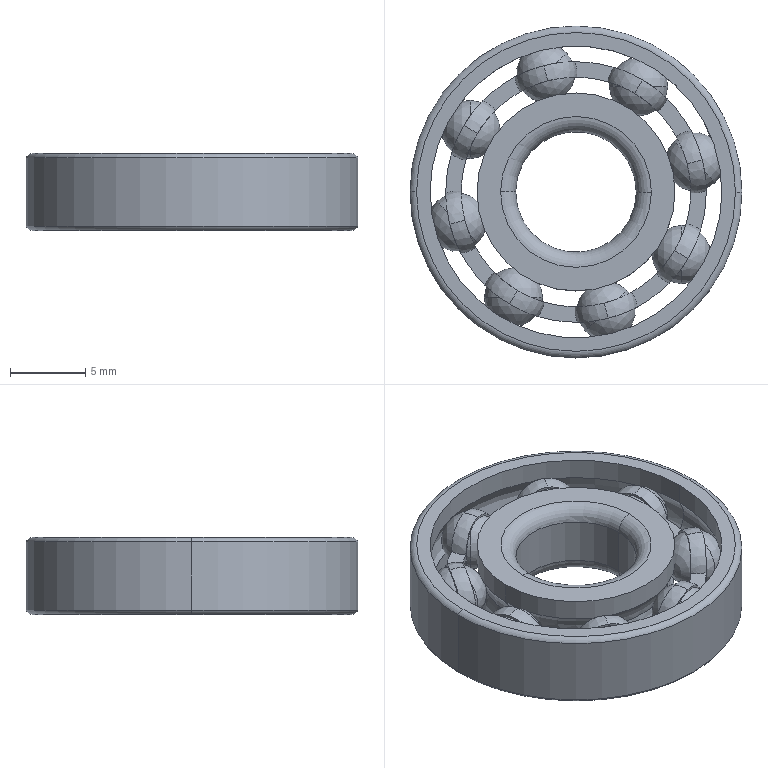Component | SolidWorks | RollerBearing22_8Thickness7-1 | 11 solids | 114 faces | volume 1064 mm3 | sphere 64 | plane 20 | cylinder 16 | torus 14 | commonest cylinder face diameters 19.337 x4 13.122 x4 22 x2 8 x2 17.266 x2 15.194 x2